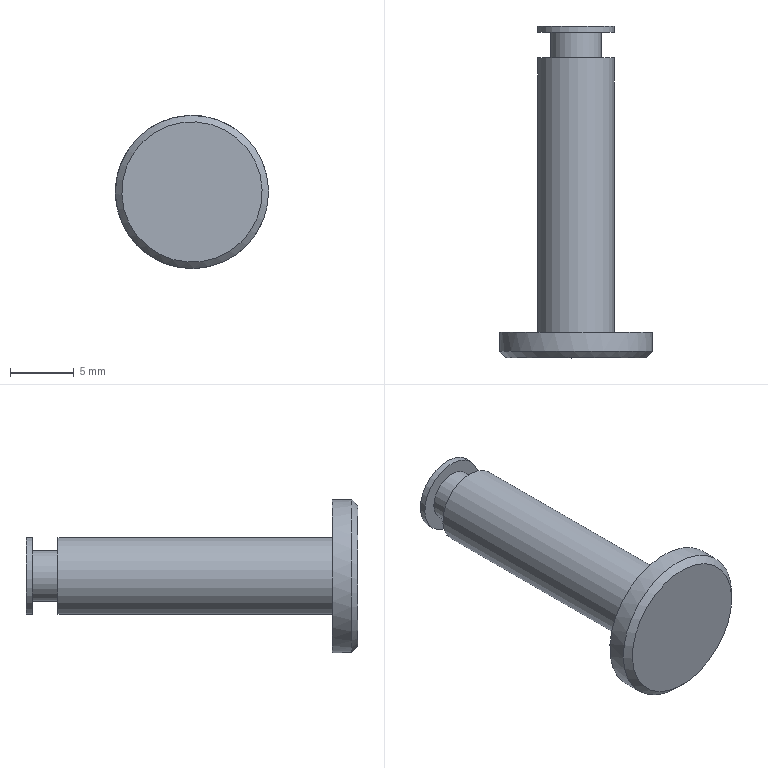Component | NX | CLHKJG_11_PIVOT_PIN | 1 solid | 10 faces | box 12 x 26 x 12 mm | volume 869 mm3 | plane 5 | cylinder 4 | cone 1 | commonest cylinder face diameters 6 x2 12 x1 4 x1
STEP:
#1=CARTESIAN_POINT('',(0.,0.,0.));
#2=DIRECTION('',(0.,0.,1.));
#3=DIRECTION('',(1.,0.,0.));
#4=AXIS2_PLACEMENT_3D('',#1,#2,#3);
#5=CARTESIAN_POINT('',(-331.441,94.165,-93.765));
#6=VERTEX_POINT('',#5);
#7=CARTESIAN_POINT('',(-334.398,94.165,-93.259));
#8=DIRECTION('',(0.,1.,0.));
#9=DIRECTION('',(0.9857,0.,-0.1686));
#10=AXIS2_PLACEMENT_3D('',#7,#8,#9);
#11=CIRCLE('',#10,3.);
#12=CARTESIAN_POINT('',(-334.398,94.165,-93.259));
#13=DIRECTION('',(0.,1.,0.));
#14=DIRECTION('',(0.9857,0.,-0.1686));
#15=AXIS2_PLACEMENT_3D('',#12,#13,#14);
#16=PLANE('',#15);
#17=CARTESIAN_POINT('',(0.,0.));
#18=DIRECTION('',(1.,0.));
#19=AXIS2_PLACEMENT_2D('',#17,#18);
#20=CIRCLE('',#19,3.);
#21=(GEOMETRIC_REPRESENTATION_CONTEXT(2)PARAMETRIC_REPRESENTATION_CONTEXT()REPRESENTATION_CONTEXT('',''));
#22=DEFINITIONAL_REPRESENTATION('',(#20),#21);
#23=PCURVE('',#16,#22);
#24=CARTESIAN_POINT('',(-334.398,94.165,-93.259));
#25=DIRECTION('',(0.,1.,0.));
#26=DIRECTION('',(0.9857,0.,-0.1686));
#27=AXIS2_PLACEMENT_3D('',#24,#25,#26);
#28=CYLINDRICAL_SURFACE('',#27,3.);
#29=CARTESIAN_POINT('',(0.,0.));
#30=DIRECTION('',(1.,0.));
#31=VECTOR('',#30,1.);
#32=LINE('',#29,#31);
#33=(GEOMETRIC_REPRESENTATION_CONTEXT(2)PARAMETRIC_REPRESENTATION_CONTEXT()REPRESENTATION_CONTEXT('',''));
#34=DEFINITIONAL_REPRESENTATION('',(#32),#33);
#35=PCURVE('',#28,#34);
#36=SURFACE_CURVE('',#11,(#23,#35),.PCURVE_S1.);
#37=EDGE_CURVE('',#6,#6,#36,.T.);
#38=ORIENTED_EDGE('',*,*,#37,.F.);
#39=EDGE_LOOP('',(#38));
#40=FACE_BOUND('',#39,.T.);
#41=CARTESIAN_POINT('',(-328.484,94.165,-94.271));
#42=VERTEX_POINT('',#41);
#43=CARTESIAN_POINT('',(-334.398,94.165,-93.259));
#44=DIRECTION('',(0.,-1.,0.));
#45=DIRECTION('',(0.9857,0.,-0.1686));
#46=AXIS2_PLACEMENT_3D('',#43,#44,#45);
#47=CIRCLE('',#46,6.);
#48=CARTESIAN_POINT('',(6.,0.));
#49=CARTESIAN_POINT('',(6.,-10.392));
#50=CARTESIAN_POINT('',(-3.,-5.196));
#51=CARTESIAN_POINT('',(-12.,-0.));
#52=CARTESIAN_POINT('',(-3.,5.196));
#53=CARTESIAN_POINT('',(6.,10.392));
#54=CARTESIAN_POINT('',(6.,0.));
#55=(BOUNDED_CURVE()B_SPLINE_CURVE(2,(#48,#49,#50,#51,#52,#53,#54),.UNSPECIFIED.,.T.,.F.)B_SPLINE_CURVE_WITH_KNOTS((1,2,2,2,2,1),(-2.094,0.,2.094,4.189,6.283,8.378),.UNSPECIFIED.)CURVE()GEOMETRIC_REPRESENTATION_ITEM()RATIONAL_B_SPLINE_CURVE((1.,0.5,1.,0.5,1.,0.5,1.))REPRESENTATION_ITEM(''));
#56=(GEOMETRIC_REPRESENTATION_CONTEXT(2)PARAMETRIC_REPRESENTATION_CONTEXT()REPRESENTATION_CONTEXT('',''));
#57=DEFINITIONAL_REPRESENTATION('',(#55),#56);
#58=PCURVE('',#16,#57);
#59=CARTESIAN_POINT('',(-334.398,92.165,-93.259));
#60=DIRECTION('',(0.,1.,0.));
#61=DIRECTION('',(0.9857,0.,-0.1686));
#62=AXIS2_PLACEMENT_3D('',#59,#60,#61);
#63=CYLINDRICAL_SURFACE('',#62,6.);
#64=CARTESIAN_POINT('',(6.283,2.));
#65=DIRECTION('',(-1.,0.));
#66=VECTOR('',#65,1.);
#67=LINE('',#64,#66);
#68=(GEOMETRIC_REPRESENTATION_CONTEXT(2)PARAMETRIC_REPRESENTATION_CONTEXT()REPRESENTATION_CONTEXT('',''));
#69=DEFINITIONAL_REPRESENTATION('',(#67),#68);
#70=PCURVE('',#63,#69);
#71=SURFACE_CURVE('',#47,(#58,#70),.PCURVE_S1.);
#72=EDGE_CURVE('',#42,#42,#71,.T.);
#73=ORIENTED_EDGE('',*,*,#72,.F.);
#74=EDGE_LOOP('',(#73));
#75=FACE_BOUND('',#74,.T.);
#76=ADVANCED_FACE('',(#40,#75),#16,.T.);
#77=CARTESIAN_POINT('',(-339.82,92.165,-92.331));
#78=VERTEX_POINT('',#77);
#79=CARTESIAN_POINT('',(-334.398,92.165,-93.259));
#80=DIRECTION('',(0.,-1.,0.));
#81=DIRECTION('',(-0.9857,0.,0.1686));
#82=AXIS2_PLACEMENT_3D('',#79,#80,#81);
#83=CIRCLE('',#82,5.5);
#84=CARTESIAN_POINT('',(-334.398,92.165,-93.259));
#85=DIRECTION('',(0.,-1.,0.));
#86=DIRECTION('',(-0.9857,0.,0.1686));
#87=AXIS2_PLACEMENT_3D('',#84,#85,#86);
#88=PLANE('',#87);
#89=CARTESIAN_POINT('',(0.,0.));
#90=DIRECTION('',(1.,0.));
#91=AXIS2_PLACEMENT_2D('',#89,#90);
#92=CIRCLE('',#91,5.5);
#93=(GEOMETRIC_REPRESENTATION_CONTEXT(2)PARAMETRIC_REPRESENTATION_CONTEXT()REPRESENTATION_CONTEXT('',''));
#94=DEFINITIONAL_REPRESENTATION('',(#92),#93);
#95=PCURVE('',#88,#94);
#96=CARTESIAN_POINT('',(-334.398,92.665,-93.259));
#97=DIRECTION('',(0.,1.,0.));
#98=DIRECTION('',(0.9857,0.,-0.1686));
#99=AXIS2_PLACEMENT_3D('',#96,#97,#98);
#100=CONICAL_SURFACE('',#99,6.,0.7854);
#101=CARTESIAN_POINT('',(9.425,-0.5));
#102=DIRECTION('',(-1.,0.));
#103=VECTOR('',#102,1.);
#104=LINE('',#101,#103);
#105=(GEOMETRIC_REPRESENTATION_CONTEXT(2)PARAMETRIC_REPRESENTATION_CONTEXT()REPRESENTATION_CONTEXT('',''));
#106=DEFINITIONAL_REPRESENTATION('',(#104),#105);
#107=PCURVE('',#100,#106);
#108=SURFACE_CURVE('',#83,(#95,#107),.PCURVE_S1.);
#109=EDGE_CURVE('',#78,#78,#108,.T.);
#110=ORIENTED_EDGE('',*,*,#109,.T.);
#111=EDGE_LOOP('',(#110));
#112=FACE_BOUND('',#111,.T.);
#113=ADVANCED_FACE('',(#112),#88,.T.);
#114=CARTESIAN_POINT('',(-340.312,92.665,-92.247));
#115=VERTEX_POINT('',#114);
#116=CARTESIAN_POINT('',(-328.484,92.665,-94.271));
#117=VERTEX_POINT('',#116);
#118=CARTESIAN_POINT('',(-334.398,92.665,-93.259));
#119=DIRECTION('',(0.,1.,0.));
#120=DIRECTION('',(-0.9857,0.,0.1686));
#121=AXIS2_PLACEMENT_3D('',#118,#119,#120);
#122=CIRCLE('',#121,6.);
#123=CARTESIAN_POINT('',(3.142,0.5));
#124=DIRECTION('',(1.,0.));
#125=VECTOR('',#124,1.);
#126=LINE('',#123,#125);
#127=(GEOMETRIC_REPRESENTATION_CONTEXT(2)PARAMETRIC_REPRESENTATION_CONTEXT()REPRESENTATION_CONTEXT('',''));
#128=DEFINITIONAL_REPRESENTATION('',(#126),#127);
#129=PCURVE('',#63,#128);
#130=CARTESIAN_POINT('',(3.142,0.));
#131=DIRECTION('',(1.,-0.));
#132=VECTOR('',#131,1.);
#133=LINE('',#130,#132);
#134=(GEOMETRIC_REPRESENTATION_CONTEXT(2)PARAMETRIC_REPRESENTATION_CONTEXT()REPRESENTATION_CONTEXT('',''));
#135=DEFINITIONAL_REPRESENTATION('',(#133),#134);
#136=PCURVE('',#100,#135);
#137=SURFACE_CURVE('',#122,(#129,#136),.PCURVE_S1.);
#138=EDGE_CURVE('',#115,#117,#137,.T.);
#139=ORIENTED_EDGE('',*,*,#138,.T.);
#140=CARTESIAN_POINT('',(-328.484,92.665,-94.271));
#141=CARTESIAN_POINT('',(-328.484,94.165,-94.271));
#142=B_SPLINE_CURVE_WITH_KNOTS('',1,(#140,#141),.UNSPECIFIED.,.F.,.F.,(2,2),(0.5,2.),.PIECEWISE_BEZIER_KNOTS.);
#143=CARTESIAN_POINT('',(6.283,0.));
#144=DIRECTION('',(0.,1.));
#145=VECTOR('',#144,1.);
#146=LINE('',#143,#145);
#147=(GEOMETRIC_REPRESENTATION_CONTEXT(2)PARAMETRIC_REPRESENTATION_CONTEXT()REPRESENTATION_CONTEXT('',''));
#148=DEFINITIONAL_REPRESENTATION('',(#146),#147);
#149=PCURVE('',#63,#148);
#150=CARTESIAN_POINT('',(0.,0.));
#151=DIRECTION('',(0.,1.));
#152=VECTOR('',#151,1.);
#153=LINE('',#150,#152);
#154=(GEOMETRIC_REPRESENTATION_CONTEXT(2)PARAMETRIC_REPRESENTATION_CONTEXT()REPRESENTATION_CONTEXT('',''));
#155=DEFINITIONAL_REPRESENTATION('',(#153),#154);
#156=PCURVE('',#63,#155);
#157=SEAM_CURVE('',#142,(#149,#156),.PCURVE_S1.);
#158=EDGE_CURVE('',#117,#42,#157,.T.);
#159=ORIENTED_EDGE('',*,*,#158,.T.);
#160=ORIENTED_EDGE('',*,*,#72,.T.);
#161=ORIENTED_EDGE('',*,*,#158,.F.);
#162=CARTESIAN_POINT('',(-334.398,92.665,-93.259));
#163=DIRECTION('',(0.,1.,0.));
#164=DIRECTION('',(-0.9857,0.,0.1686));
#165=AXIS2_PLACEMENT_3D('',#162,#163,#164);
#166=CIRCLE('',#165,6.);
#167=CARTESIAN_POINT('',(-3.142,0.5));
#168=DIRECTION('',(1.,0.));
#169=VECTOR('',#168,1.);
#170=LINE('',#167,#169);
#171=(GEOMETRIC_REPRESENTATION_CONTEXT(2)PARAMETRIC_REPRESENTATION_CONTEXT()REPRESENTATION_CONTEXT('',''));
#172=DEFINITIONAL_REPRESENTATION('',(#170),#171);
#173=PCURVE('',#63,#172);
#174=CARTESIAN_POINT('',(3.142,-0.));
#175=DIRECTION('',(1.,0.));
#176=VECTOR('',#175,1.);
#177=LINE('',#174,#176);
#178=(GEOMETRIC_REPRESENTATION_CONTEXT(2)PARAMETRIC_REPRESENTATION_CONTEXT()REPRESENTATION_CONTEXT('',''));
#179=DEFINITIONAL_REPRESENTATION('',(#177),#178);
#180=PCURVE('',#100,#179);
#181=SURFACE_CURVE('',#166,(#173,#180),.PCURVE_S1.);
#182=EDGE_CURVE('',#117,#115,#181,.T.);
#183=ORIENTED_EDGE('',*,*,#182,.T.);
#184=EDGE_LOOP('',(#139,#159,#160,#161,#183));
#185=FACE_BOUND('',#184,.T.);
#186=ADVANCED_FACE('',(#185),#63,.T.);
#187=CARTESIAN_POINT('',(-332.427,115.665,-93.596));
#188=VERTEX_POINT('',#187);
#189=CARTESIAN_POINT('',(-334.398,115.665,-93.259));
#190=DIRECTION('',(0.,1.,0.));
#191=DIRECTION('',(0.9857,0.,-0.1686));
#192=AXIS2_PLACEMENT_3D('',#189,#190,#191);
#193=CIRCLE('',#192,2.);
#194=CARTESIAN_POINT('',(-334.398,115.665,-93.259));
#195=DIRECTION('',(0.,1.,0.));
#196=DIRECTION('',(0.9857,0.,-0.1686));
#197=AXIS2_PLACEMENT_3D('',#194,#195,#196);
#198=PLANE('',#197);
#199=CARTESIAN_POINT('',(0.,0.));
#200=DIRECTION('',(1.,0.));
#201=AXIS2_PLACEMENT_2D('',#199,#200);
#202=CIRCLE('',#201,2.);
#203=(GEOMETRIC_REPRESENTATION_CONTEXT(2)PARAMETRIC_REPRESENTATION_CONTEXT()REPRESENTATION_CONTEXT('',''));
#204=DEFINITIONAL_REPRESENTATION('',(#202),#203);
#205=PCURVE('',#198,#204);
#206=CARTESIAN_POINT('',(-334.398,115.665,-93.259));
#207=DIRECTION('',(0.,1.,0.));
#208=DIRECTION('',(0.9857,0.,-0.1686));
#209=AXIS2_PLACEMENT_3D('',#206,#207,#208);
#210=CYLINDRICAL_SURFACE('',#209,2.);
#211=CARTESIAN_POINT('',(0.,0.));
#212=DIRECTION('',(1.,0.));
#213=VECTOR('',#212,1.);
#214=LINE('',#211,#213);
#215=(GEOMETRIC_REPRESENTATION_CONTEXT(2)PARAMETRIC_REPRESENTATION_CONTEXT()REPRESENTATION_CONTEXT('',''));
#216=DEFINITIONAL_REPRESENTATION('',(#214),#215);
#217=PCURVE('',#210,#216);
#218=SURFACE_CURVE('',#193,(#205,#217),.PCURVE_S1.);
#219=EDGE_CURVE('',#188,#188,#218,.T.);
#220=ORIENTED_EDGE('',*,*,#219,.F.);
#221=EDGE_LOOP('',(#220));
#222=FACE_BOUND('',#221,.T.);
#223=CARTESIAN_POINT('',(-331.441,115.665,-93.765));
#224=VERTEX_POINT('',#223);
#225=CARTESIAN_POINT('',(-334.398,115.665,-93.259));
#226=DIRECTION('',(0.,-1.,0.));
#227=DIRECTION('',(0.9857,0.,-0.1686));
#228=AXIS2_PLACEMENT_3D('',#225,#226,#227);
#229=CIRCLE('',#228,3.);
#230=CARTESIAN_POINT('',(3.,0.));
#231=CARTESIAN_POINT('',(3.,-5.196));
#232=CARTESIAN_POINT('',(-1.5,-2.598));
#233=CARTESIAN_POINT('',(-6.,-0.));
#234=CARTESIAN_POINT('',(-1.5,2.598));
#235=CARTESIAN_POINT('',(3.,5.196));
#236=CARTESIAN_POINT('',(3.,0.));
#237=(BOUNDED_CURVE()B_SPLINE_CURVE(2,(#230,#231,#232,#233,#234,#235,#236),.UNSPECIFIED.,.T.,.F.)B_SPLINE_CURVE_WITH_KNOTS((1,2,2,2,2,1),(-2.094,0.,2.094,4.189,6.283,8.378),.UNSPECIFIED.)CURVE()GEOMETRIC_REPRESENTATION_ITEM()RATIONAL_B_SPLINE_CURVE((1.,0.5,1.,0.5,1.,0.5,1.))REPRESENTATION_ITEM(''));
#238=(GEOMETRIC_REPRESENTATION_CONTEXT(2)PARAMETRIC_REPRESENTATION_CONTEXT()REPRESENTATION_CONTEXT('',''));
#239=DEFINITIONAL_REPRESENTATION('',(#237),#238);
#240=PCURVE('',#198,#239);
#241=CARTESIAN_POINT('',(6.283,21.5));
#242=DIRECTION('',(-1.,0.));
#243=VECTOR('',#242,1.);
#244=LINE('',#241,#243);
#245=(GEOMETRIC_REPRESENTATION_CONTEXT(2)PARAMETRIC_REPRESENTATION_CONTEXT()REPRESENTATION_CONTEXT('',''));
#246=DEFINITIONAL_REPRESENTATION('',(#244),#245);
#247=PCURVE('',#28,#246);
#248=SURFACE_CURVE('',#229,(#240,#247),.PCURVE_S1.);
#249=EDGE_CURVE('',#224,#224,#248,.T.);
#250=ORIENTED_EDGE('',*,*,#249,.F.);
#251=EDGE_LOOP('',(#250));
#252=FACE_BOUND('',#251,.T.);
#253=ADVANCED_FACE('',(#222,#252),#198,.T.);
#254=ORIENTED_EDGE('',*,*,#249,.T.);
#255=CARTESIAN_POINT('',(-331.441,94.165,-93.765));
#256=CARTESIAN_POINT('',(-331.441,115.665,-93.765));
#257=B_SPLINE_CURVE_WITH_KNOTS('',1,(#255,#256),.UNSPECIFIED.,.F.,.F.,(2,2),(0.,21.5),.PIECEWISE_BEZIER_KNOTS.);
#258=CARTESIAN_POINT('',(0.,0.));
#259=DIRECTION('',(0.,1.));
#260=VECTOR('',#259,1.);
#261=LINE('',#258,#260);
#262=(GEOMETRIC_REPRESENTATION_CONTEXT(2)PARAMETRIC_REPRESENTATION_CONTEXT()REPRESENTATION_CONTEXT('',''));
#263=DEFINITIONAL_REPRESENTATION('',(#261),#262);
#264=PCURVE('',#28,#263);
#265=CARTESIAN_POINT('',(6.283,0.));
#266=DIRECTION('',(0.,1.));
#267=VECTOR('',#266,1.);
#268=LINE('',#265,#267);
#269=(GEOMETRIC_REPRESENTATION_CONTEXT(2)PARAMETRIC_REPRESENTATION_CONTEXT()REPRESENTATION_CONTEXT('',''));
#270=DEFINITIONAL_REPRESENTATION('',(#268),#269);
#271=PCURVE('',#28,#270);
#272=SEAM_CURVE('',#257,(#264,#271),.PCURVE_S1.);
#273=EDGE_CURVE('',#6,#224,#272,.T.);
#274=ORIENTED_EDGE('',*,*,#273,.F.);
#275=ORIENTED_EDGE('',*,*,#37,.T.);
#276=ORIENTED_EDGE('',*,*,#273,.T.);
#277=EDGE_LOOP('',(#254,#274,#275,#276));
#278=FACE_BOUND('',#277,.T.);
#279=ADVANCED_FACE('',(#278),#28,.T.);
#280=CARTESIAN_POINT('',(-332.427,117.665,-93.596));
#281=VERTEX_POINT('',#280);
#282=CARTESIAN_POINT('',(-334.398,117.665,-93.259));
#283=DIRECTION('',(0.,-1.,0.));
#284=DIRECTION('',(0.9857,0.,-0.1686));
#285=AXIS2_PLACEMENT_3D('',#282,#283,#284);
#286=CIRCLE('',#285,2.);
#287=CARTESIAN_POINT('',(6.283,2.));
#288=DIRECTION('',(-1.,0.));
#289=VECTOR('',#288,1.);
#290=LINE('',#287,#289);
#291=(GEOMETRIC_REPRESENTATION_CONTEXT(2)PARAMETRIC_REPRESENTATION_CONTEXT()REPRESENTATION_CONTEXT('',''));
#292=DEFINITIONAL_REPRESENTATION('',(#290),#291);
#293=PCURVE('',#210,#292);
#294=CARTESIAN_POINT('',(-334.398,117.665,-93.259));
#295=DIRECTION('',(0.,-1.,0.));
#296=DIRECTION('',(-0.9857,0.,0.1686));
#297=AXIS2_PLACEMENT_3D('',#294,#295,#296);
#298=PLANE('',#297);
#299=CARTESIAN_POINT('',(0.,0.));
#300=DIRECTION('',(-1.,0.));
#301=AXIS2_PLACEMENT_2D('',#299,#300);
#302=CIRCLE('',#301,2.);
#303=(GEOMETRIC_REPRESENTATION_CONTEXT(2)PARAMETRIC_REPRESENTATION_CONTEXT()REPRESENTATION_CONTEXT('',''));
#304=DEFINITIONAL_REPRESENTATION('',(#302),#303);
#305=PCURVE('',#298,#304);
#306=SURFACE_CURVE('',#286,(#293,#305),.PCURVE_S1.);
#307=EDGE_CURVE('',#281,#281,#306,.T.);
#308=ORIENTED_EDGE('',*,*,#307,.T.);
#309=CARTESIAN_POINT('',(-332.427,115.665,-93.596));
#310=CARTESIAN_POINT('',(-332.427,117.665,-93.596));
#311=B_SPLINE_CURVE_WITH_KNOTS('',1,(#309,#310),.UNSPECIFIED.,.F.,.F.,(2,2),(0.,2.),.PIECEWISE_BEZIER_KNOTS.);
#312=CARTESIAN_POINT('',(0.,0.));
#313=DIRECTION('',(0.,1.));
#314=VECTOR('',#313,1.);
#315=LINE('',#312,#314);
#316=(GEOMETRIC_REPRESENTATION_CONTEXT(2)PARAMETRIC_REPRESENTATION_CONTEXT()REPRESENTATION_CONTEXT('',''));
#317=DEFINITIONAL_REPRESENTATION('',(#315),#316);
#318=PCURVE('',#210,#317);
#319=CARTESIAN_POINT('',(6.283,0.));
#320=DIRECTION('',(0.,1.));
#321=VECTOR('',#320,1.);
#322=LINE('',#319,#321);
#323=(GEOMETRIC_REPRESENTATION_CONTEXT(2)PARAMETRIC_REPRESENTATION_CONTEXT()REPRESENTATION_CONTEXT('',''));
#324=DEFINITIONAL_REPRESENTATION('',(#322),#323);
#325=PCURVE('',#210,#324);
#326=SEAM_CURVE('',#311,(#318,#325),.PCURVE_S1.);
#327=EDGE_CURVE('',#188,#281,#326,.T.);
#328=ORIENTED_EDGE('',*,*,#327,.F.);
#329=ORIENTED_EDGE('',*,*,#219,.T.);
#330=ORIENTED_EDGE('',*,*,#327,.T.);
#331=EDGE_LOOP('',(#308,#328,#329,#330));
#332=FACE_BOUND('',#331,.T.);
#333=ADVANCED_FACE('',(#332),#210,.T.);
#334=CARTESIAN_POINT('',(-331.441,118.165,-93.765));
#335=VERTEX_POINT('',#334);
#336=CARTESIAN_POINT('',(-334.398,118.165,-93.259));
#337=DIRECTION('',(0.,-1.,0.));
#338=DIRECTION('',(0.9857,0.,-0.1686));
#339=AXIS2_PLACEMENT_3D('',#336,#337,#338);
#340=CIRCLE('',#339,3.);
#341=CARTESIAN_POINT('',(-334.398,118.165,-93.259));
#342=DIRECTION('',(0.,1.,0.));
#343=DIRECTION('',(0.9857,0.,-0.1686));
#344=AXIS2_PLACEMENT_3D('',#341,#342,#343);
#345=PLANE('',#344);
#346=CARTESIAN_POINT('',(3.,0.));
#347=CARTESIAN_POINT('',(3.,-5.196));
#348=CARTESIAN_POINT('',(-1.5,-2.598));
#349=CARTESIAN_POINT('',(-6.,-0.));
#350=CARTESIAN_POINT('',(-1.5,2.598));
#351=CARTESIAN_POINT('',(3.,5.196));
#352=CARTESIAN_POINT('',(3.,0.));
#353=(BOUNDED_CURVE()B_SPLINE_CURVE(2,(#346,#347,#348,#349,#350,#351,#352),.UNSPECIFIED.,.T.,.F.)B_SPLINE_CURVE_WITH_KNOTS((1,2,2,2,2,1),(-2.094,0.,2.094,4.189,6.283,8.378),.UNSPECIFIED.)CURVE()GEOMETRIC_REPRESENTATION_ITEM()RATIONAL_B_SPLINE_CURVE((1.,0.5,1.,0.5,1.,0.5,1.))REPRESENTATION_ITEM(''));
#354=(GEOMETRIC_REPRESENTATION_CONTEXT(2)PARAMETRIC_REPRESENTATION_CONTEXT()REPRESENTATION_CONTEXT('',''));
#355=DEFINITIONAL_REPRESENTATION('',(#353),#354);
#356=PCURVE('',#345,#355);
#357=CARTESIAN_POINT('',(-334.398,117.665,-93.259));
#358=DIRECTION('',(0.,1.,0.));
#359=DIRECTION('',(0.9857,0.,-0.1686));
#360=AXIS2_PLACEMENT_3D('',#357,#358,#359);
#361=CYLINDRICAL_SURFACE('',#360,3.);
#362=CARTESIAN_POINT('',(6.283,0.5));
#363=DIRECTION('',(-1.,0.));
#364=VECTOR('',#363,1.);
#365=LINE('',#362,#364);
#366=(GEOMETRIC_REPRESENTATION_CONTEXT(2)PARAMETRIC_REPRESENTATION_CONTEXT()REPRESENTATION_CONTEXT('',''));
#367=DEFINITIONAL_REPRESENTATION('',(#365),#366);
#368=PCURVE('',#361,#367);
#369=SURFACE_CURVE('',#340,(#356,#368),.PCURVE_S1.);
#370=EDGE_CURVE('',#335,#335,#369,.T.);
#371=ORIENTED_EDGE('',*,*,#370,.F.);
#372=EDGE_LOOP('',(#371));
#373=FACE_BOUND('',#372,.T.);
#374=ADVANCED_FACE('',(#373),#345,.T.);
#375=ORIENTED_EDGE('',*,*,#307,.F.);
#376=EDGE_LOOP('',(#375));
#377=FACE_BOUND('',#376,.T.);
#378=CARTESIAN_POINT('',(-331.441,117.665,-93.765));
#379=VERTEX_POINT('',#378);
#380=CARTESIAN_POINT('',(-334.398,117.665,-93.259));
#381=DIRECTION('',(0.,1.,0.));
#382=DIRECTION('',(0.9857,0.,-0.1686));
#383=AXIS2_PLACEMENT_3D('',#380,#381,#382);
#384=CIRCLE('',#383,3.);
#385=CARTESIAN_POINT('',(-3.,0.));
#386=CARTESIAN_POINT('',(-3.,5.196));
#387=CARTESIAN_POINT('',(1.5,2.598));
#388=CARTESIAN_POINT('',(6.,-0.));
#389=CARTESIAN_POINT('',(1.5,-2.598));
#390=CARTESIAN_POINT('',(-3.,-5.196));
#391=CARTESIAN_POINT('',(-3.,0.));
#392=(BOUNDED_CURVE()B_SPLINE_CURVE(2,(#385,#386,#387,#388,#389,#390,#391),.UNSPECIFIED.,.T.,.F.)B_SPLINE_CURVE_WITH_KNOTS((1,2,2,2,2,1),(-2.094,0.,2.094,4.189,6.283,8.378),.UNSPECIFIED.)CURVE()GEOMETRIC_REPRESENTATION_ITEM()RATIONAL_B_SPLINE_CURVE((1.,0.5,1.,0.5,1.,0.5,1.))REPRESENTATION_ITEM(''));
#393=(GEOMETRIC_REPRESENTATION_CONTEXT(2)PARAMETRIC_REPRESENTATION_CONTEXT()REPRESENTATION_CONTEXT('',''));
#394=DEFINITIONAL_REPRESENTATION('',(#392),#393);
#395=PCURVE('',#298,#394);
#396=CARTESIAN_POINT('',(0.,0.));
#397=DIRECTION('',(1.,0.));
#398=VECTOR('',#397,1.);
#399=LINE('',#396,#398);
#400=(GEOMETRIC_REPRESENTATION_CONTEXT(2)PARAMETRIC_REPRESENTATION_CONTEXT()REPRESENTATION_CONTEXT('',''));
#401=DEFINITIONAL_REPRESENTATION('',(#399),#400);
#402=PCURVE('',#361,#401);
#403=SURFACE_CURVE('',#384,(#395,#402),.PCURVE_S1.);
#404=EDGE_CURVE('',#379,#379,#403,.T.);
#405=ORIENTED_EDGE('',*,*,#404,.F.);
#406=EDGE_LOOP('',(#405));
#407=FACE_BOUND('',#406,.T.);
#408=ADVANCED_FACE('',(#377,#407),#298,.T.);
#409=ORIENTED_EDGE('',*,*,#370,.T.);
#410=CARTESIAN_POINT('',(-331.441,117.665,-93.765));
#411=CARTESIAN_POINT('',(-331.441,118.165,-93.765));
#412=B_SPLINE_CURVE_WITH_KNOTS('',1,(#410,#411),.UNSPECIFIED.,.F.,.F.,(2,2),(0.,0.5),.PIECEWISE_BEZIER_KNOTS.);
#413=CARTESIAN_POINT('',(0.,0.));
#414=DIRECTION('',(0.,1.));
#415=VECTOR('',#414,1.);
#416=LINE('',#413,#415);
#417=(GEOMETRIC_REPRESENTATION_CONTEXT(2)PARAMETRIC_REPRESENTATION_CONTEXT()REPRESENTATION_CONTEXT('',''));
#418=DEFINITIONAL_REPRESENTATION('',(#416),#417);
#419=PCURVE('',#361,#418);
#420=CARTESIAN_POINT('',(6.283,0.));
#421=DIRECTION('',(0.,1.));
#422=VECTOR('',#421,1.);
#423=LINE('',#420,#422);
#424=(GEOMETRIC_REPRESENTATION_CONTEXT(2)PARAMETRIC_REPRESENTATION_CONTEXT()REPRESENTATION_CONTEXT('',''));
#425=DEFINITIONAL_REPRESENTATION('',(#423),#424);
#426=PCURVE('',#361,#425);
#427=SEAM_CURVE('',#412,(#419,#426),.PCURVE_S1.);
#428=EDGE_CURVE('',#379,#335,#427,.T.);
#429=ORIENTED_EDGE('',*,*,#428,.F.);
#430=ORIENTED_EDGE('',*,*,#404,.T.);
#431=ORIENTED_EDGE('',*,*,#428,.T.);
#432=EDGE_LOOP('',(#409,#429,#430,#431));
#433=FACE_BOUND('',#432,.T.);
#434=ADVANCED_FACE('',(#433),#361,.T.);
#435=ORIENTED_EDGE('',*,*,#109,.F.);
#436=CARTESIAN_POINT('',(-339.82,92.165,-92.331));
#437=CARTESIAN_POINT('',(-340.312,92.665,-92.247));
#438=B_SPLINE_CURVE_WITH_KNOTS('',1,(#436,#437),.UNSPECIFIED.,.F.,.F.,(2,2),(-0.7071,0.),.PIECEWISE_BEZIER_KNOTS.);
#439=CARTESIAN_POINT('',(9.425,0.));
#440=DIRECTION('',(0.,1.));
#441=VECTOR('',#440,1.);
#442=LINE('',#439,#441);
#443=(GEOMETRIC_REPRESENTATION_CONTEXT(2)PARAMETRIC_REPRESENTATION_CONTEXT()REPRESENTATION_CONTEXT('',''));
#444=DEFINITIONAL_REPRESENTATION('',(#442),#443);
#445=PCURVE('',#100,#444);
#446=CARTESIAN_POINT('',(3.142,0.));
#447=DIRECTION('',(0.,1.));
#448=VECTOR('',#447,1.);
#449=LINE('',#446,#448);
#450=(GEOMETRIC_REPRESENTATION_CONTEXT(2)PARAMETRIC_REPRESENTATION_CONTEXT()REPRESENTATION_CONTEXT('',''));
#451=DEFINITIONAL_REPRESENTATION('',(#449),#450);
#452=PCURVE('',#100,#451);
#453=SEAM_CURVE('',#438,(#445,#452),.PCURVE_S1.);
#454=EDGE_CURVE('',#78,#115,#453,.T.);
#455=ORIENTED_EDGE('',*,*,#454,.T.);
#456=ORIENTED_EDGE('',*,*,#182,.F.);
#457=ORIENTED_EDGE('',*,*,#138,.F.);
#458=ORIENTED_EDGE('',*,*,#454,.F.);
#459=EDGE_LOOP('',(#435,#455,#456,#457,#458));
#460=FACE_BOUND('',#459,.T.);
#461=ADVANCED_FACE('',(#460),#100,.T.);
#462=CLOSED_SHELL('',(#76,#113,#186,#253,#279,#333,#374,#408,#434,#461));
#463=MANIFOLD_SOLID_BREP('',#462);
#464=(LENGTH_UNIT()NAMED_UNIT(*)SI_UNIT(.MILLI.,.METRE.));
#465=UNCERTAINTY_MEASURE_WITH_UNIT(LENGTH_MEASURE(0.00001),#464,'','');
#466=(NAMED_UNIT(*)PLANE_ANGLE_UNIT()SI_UNIT($,.RADIAN.));
#467=(NAMED_UNIT(*)SI_UNIT($,.STERADIAN.)SOLID_ANGLE_UNIT());
#468=(GEOMETRIC_REPRESENTATION_CONTEXT(3)GLOBAL_UNCERTAINTY_ASSIGNED_CONTEXT((#465))GLOBAL_UNIT_ASSIGNED_CONTEXT((#464,#466,#467))REPRESENTATION_CONTEXT('',''));
#469=ADVANCED_BREP_SHAPE_REPRESENTATION('',(#4,#463),#468);